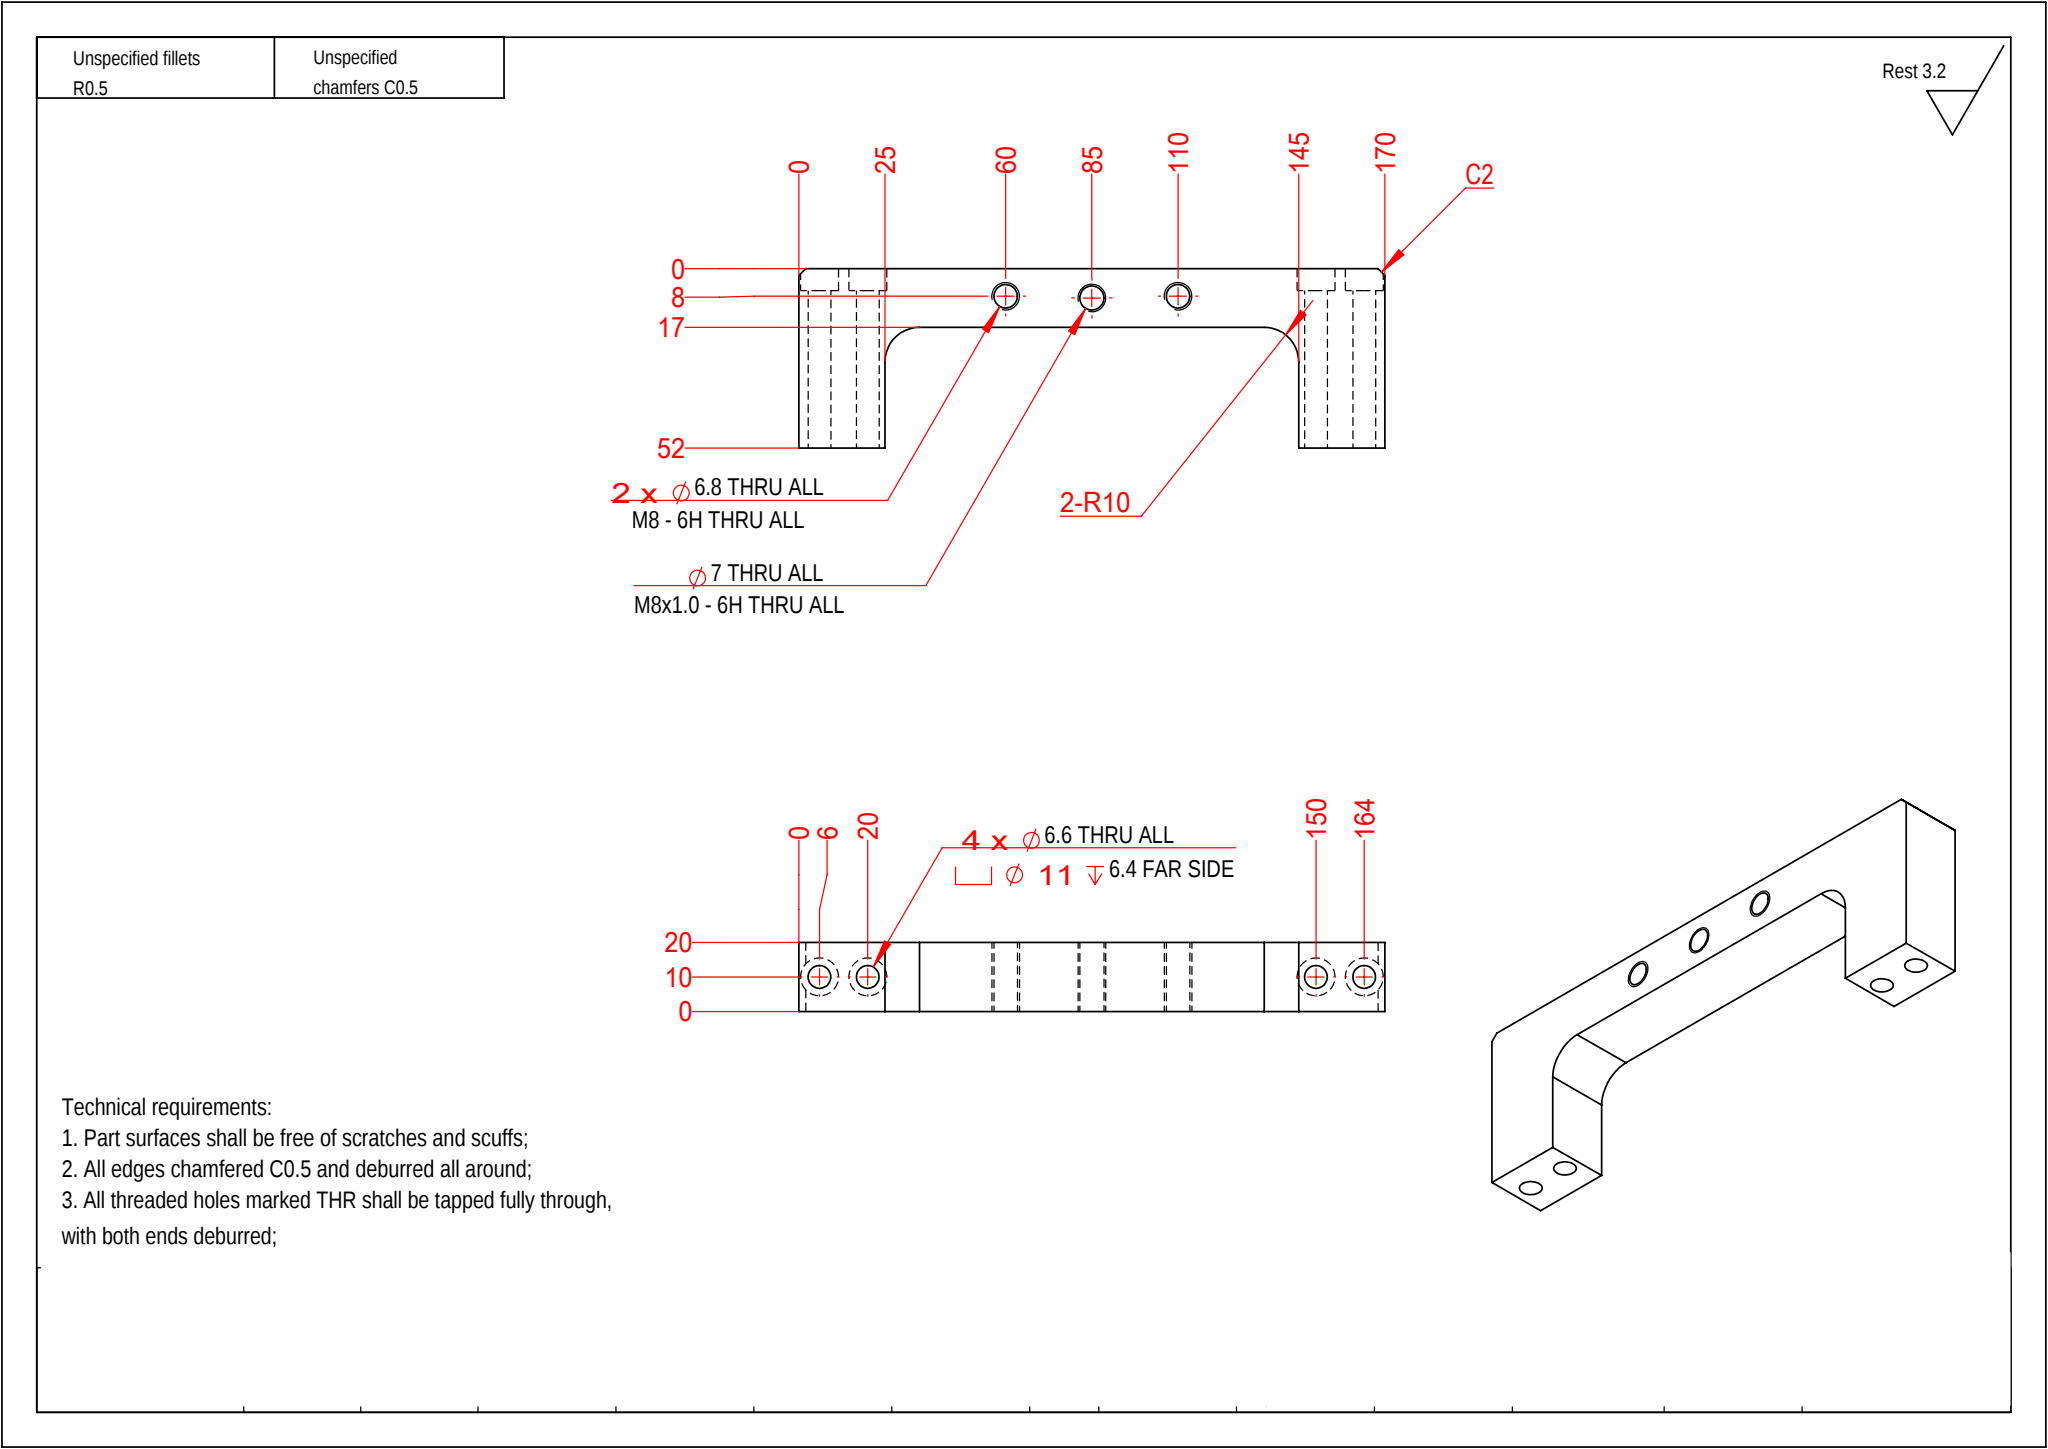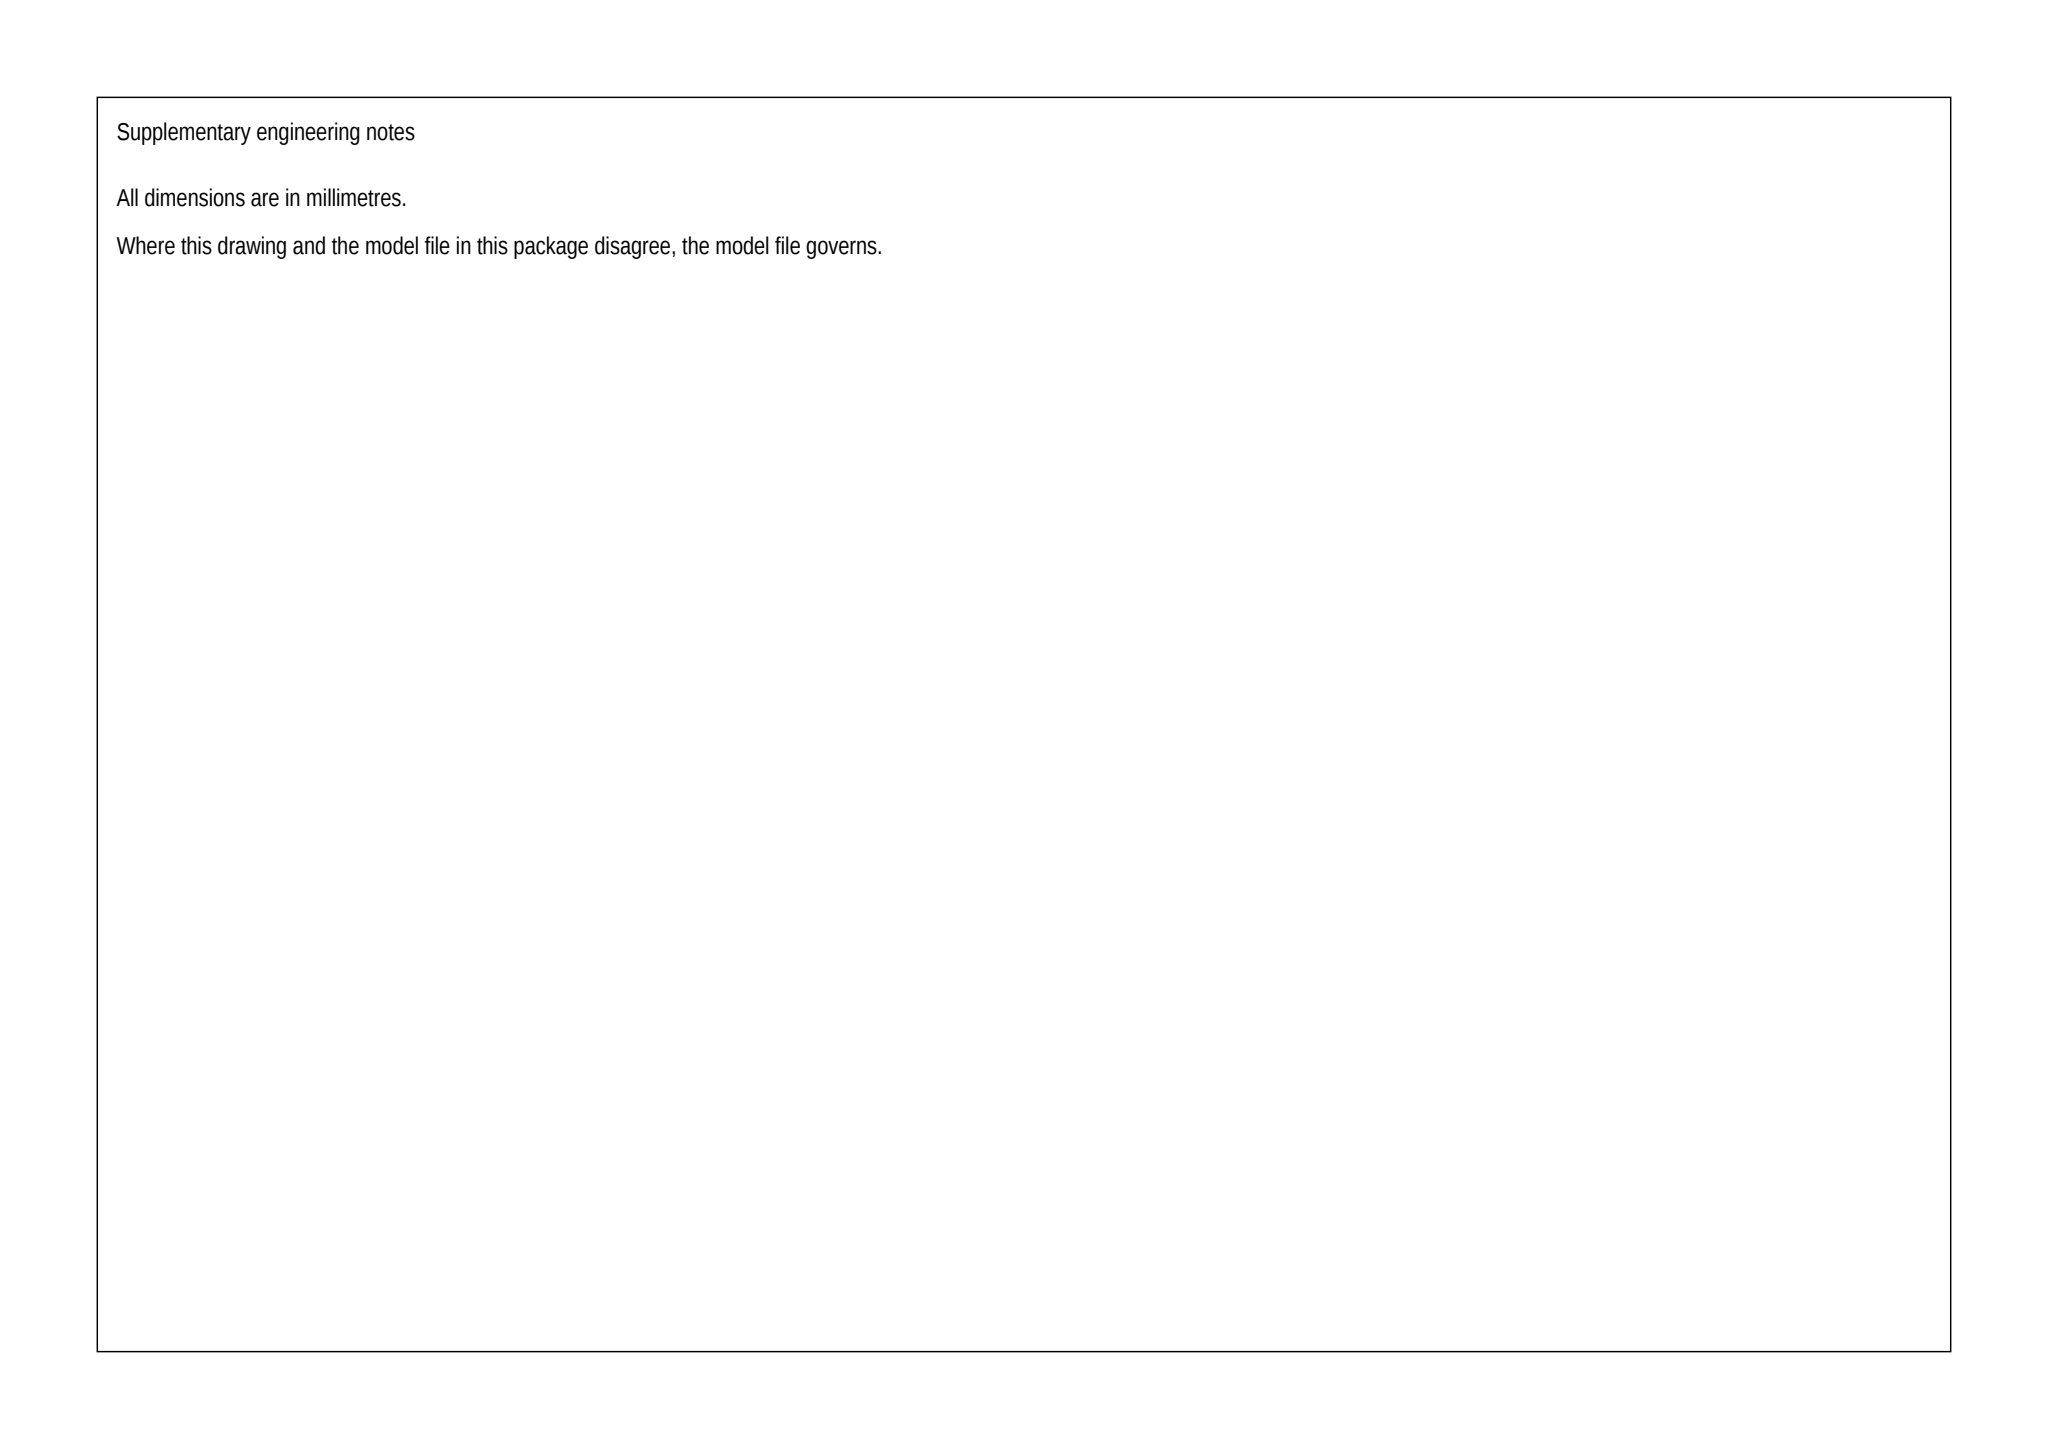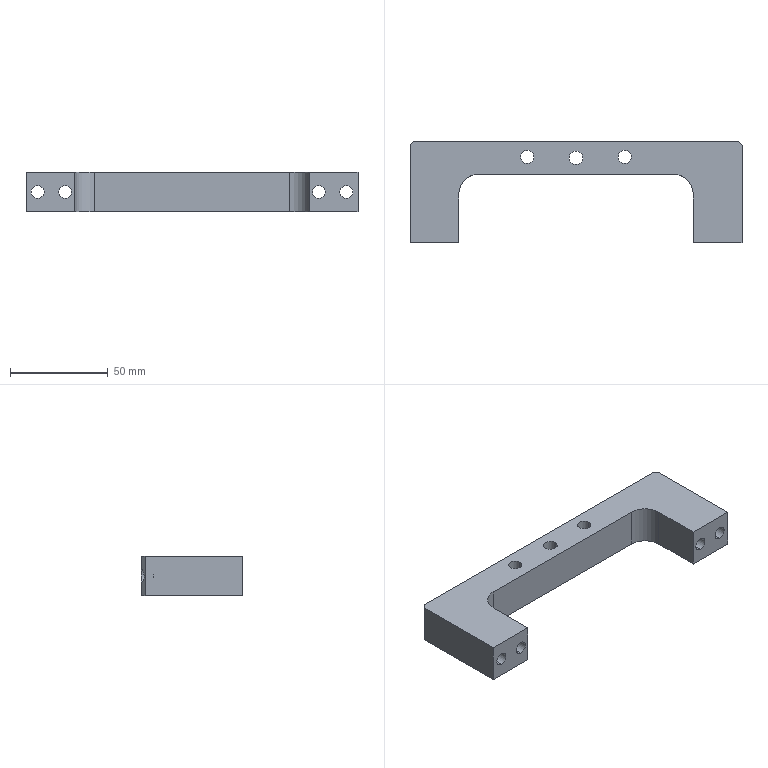Part | SolidWorks | mm | 1 solid | 40 faces | box 170 x 52 x 20 mm | volume 82692 mm3 | cylinder 24 | plane 16 | commonest cylinder face diameters 11 x8 6.6 x8 6.8 x4 7 x2 20 x2
Drawing notes:
2X M8-6H THRU (20 deep), tap drill Ø6.8; holes at X=60 and X=110, Y=44 from bbox min corner, axis parallel Z | from the solid: cylinders: [6.8,"z",[60.0,44.0,null],20.0] and [6.8,"z",[110.0,44.0,null],20.0]
4X Ø6.6 BLIND, 45.6 DEEP from Y=0 face; CBORE Ø11 DP 6.4; holes at X=6, 20, 150, 164, Z=10 from bbox min corner, axis parallel Y | from the solid: cylinders: [6.6,"y",[6/20/150/164,null,10.0],45.6] and [11.0,"y",[6/20/150/164,null,10.0],6.4]
ALL DIMENSIONS IN MILLIMETERS | from the solid: STEP model facts stated in mm
Ø7 (M8x1.0) HOLE THRU 20 DEEP: LOCATE AT X=85, Y=43.5 FROM BBOX MIN CORNER, AXIS PARALLEL Z | from the solid: cylinders: [7.0, "z", [85.0, 43.5, null], 20.0]
2X Ø6.8 TAP DRILL (M8-6H) THRU, 20 DEEP; HOLES AT X=60 AND X=110, Y=44 FROM BBOX MIN CORNER, AXIS PARALLEL Z | from the solid: cylinders dia 6.8 axis z at (60,44) and (110,44), length 20
ALL DIMENSIONS IN MILLIMETERS; PART ENVELOPE 170 x 52 x 20 | from the solid: bbox_xyz [170.0, 52.0, 20.0], origin_note positions from min corner of bbox
build123d program:
from build123d import *

# Parameters (mm, degrees)
BOSS_EXTRUDE1_DEPTH                             = 20
CHAMFER1_SIZE                                   = 2
FILLET1_R                                       = 10
M8X1_0_TAPPED_HOLE1_D                           = 7
M6_HEX_SOCKET_HEAD_CAP_SCREW_CBORE1_D           = 6.6
M6_HEX_SOCKET_HEAD_CAP_SCREW_CBORE1_CBORE_D     = 11
M6_HEX_SOCKET_HEAD_CAP_SCREW_CBORE1_CBORE_DEPTH = 6.4
M8_TAPPED_HOLE1_D                               = 6.8


with BuildPart() as part:
    # Sketch1 → Boss-Extrude1 (new body)
    with BuildSketch(Plane.XY):
        Polygon((-25, 52), (-25, 0), (0, 0), (0, 35), (120, 35), (120, 0), (145, 0), (145, 52), align=None)
    extrude(amount=BOSS_EXTRUDE1_DEPTH)

    # Chamfer1
    chamfer1_edges = [part.edges().sort_by_distance(p)[0] for p in [
        (-25, 52, 10),
        (145, 52, 10),
    ]]
    chamfer(chamfer1_edges, length=CHAMFER1_SIZE)

    # Fillet1
    fillet1_edges = [part.edges().sort_by_distance(p)[0] for p in [
        (120, 35, 10),
        (0, 35, 10),
    ]]
    fillet(fillet1_edges, radius=FILLET1_R)

    # M8x1.0 Tapped Hole1 (through all)
    with Locations(Plane.XY.offset(20)):
        with Locations((60, 43.5)):
            Hole(M8X1_0_TAPPED_HOLE1_D / 2)

    # M6 Hex Socket Head Cap Screw CBORE1 (through all)
    with Locations(Plane(origin=(0, 52, 0), x_dir=(1, 0, 0), z_dir=(0, 1, 0))):
        with Locations((-5, -10), (-19, -10), (139, -10), (125, -10)):
            CounterBoreHole(M6_HEX_SOCKET_HEAD_CAP_SCREW_CBORE1_D / 2, M6_HEX_SOCKET_HEAD_CAP_SCREW_CBORE1_CBORE_D / 2, M6_HEX_SOCKET_HEAD_CAP_SCREW_CBORE1_CBORE_DEPTH)

    # M8 Tapped Hole1 (through all)
    with Locations(Plane.XY.offset(20)):
        with Locations((35, 44), (85, 44)):
            Hole(M8_TAPPED_HOLE1_D / 2)


solid = part.part